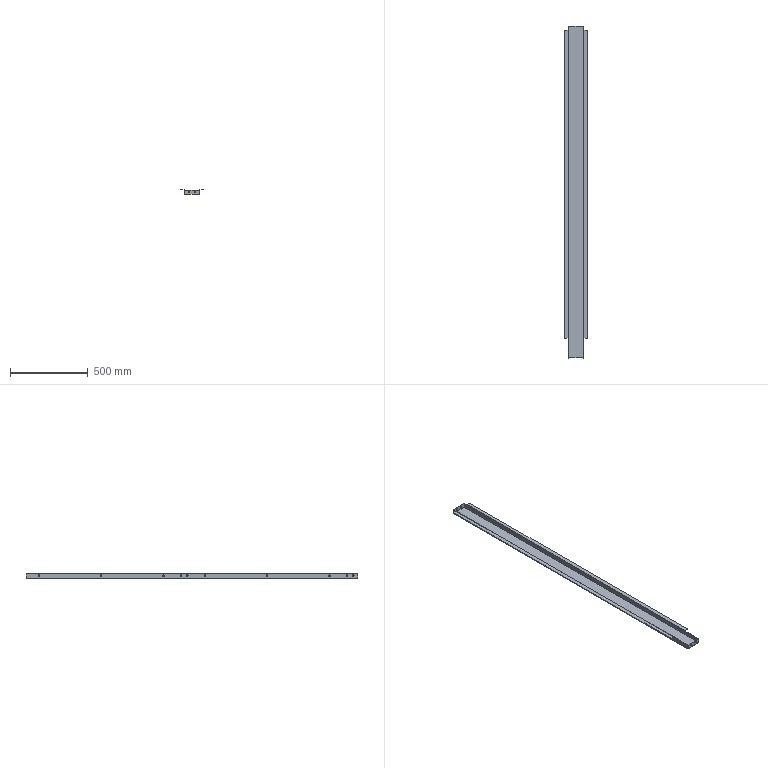Component | SolidWorks | 18RearMiddleColumn-2 | 1 solid | 110 faces | volume 869045 mm3 | cylinder 60 | plane 50 | commonest cylinder face diameters 10 x48 6 x6 2 x6